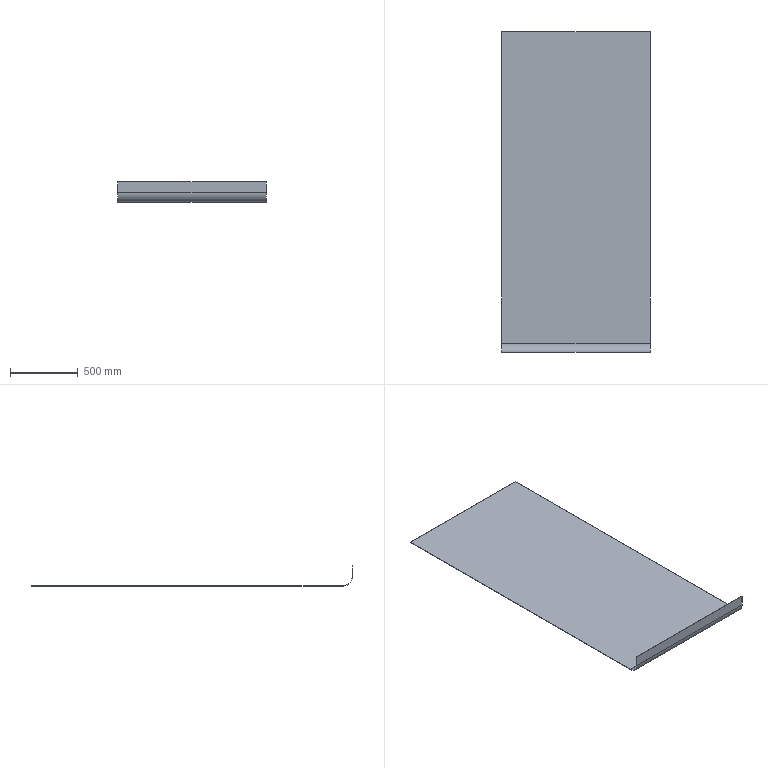Component | SolidWorks | C-SideAluminumHousingAssembly-1_C-SideAluminumCasing1-1 | 1 solid | 14 faces | box 1100 x 2375.5 x 149.5 mm | volume 8226287 mm3 | plane 12 | cylinder 2 | commonest cylinder face diameters 139 x1 133 x1
STEP:
#1=COLOUR_RGB('',0.7922,0.8196,0.9333);
#2=FILL_AREA_STYLE_COLOUR('',#1);
#3=FILL_AREA_STYLE('',(#2));
#4=SURFACE_STYLE_FILL_AREA(#3);
#5=SURFACE_SIDE_STYLE('',(#4));
#6=SURFACE_STYLE_USAGE(.BOTH.,#5);
#7=PRESENTATION_STYLE_ASSIGNMENT((#6));
#8=CARTESIAN_POINT('',(43.307,0.,-0.1181));
#9=VERTEX_POINT('',#8);
#10=CARTESIAN_POINT('',(43.307,0.,0.));
#11=VERTEX_POINT('',#10);
#12=CARTESIAN_POINT('',(43.307,0.,0.));
#13=DIRECTION('',(0.,0.,1.));
#14=VECTOR('',#13,39.37);
#15=LINE('',#12,#14);
#16=EDGE_CURVE('',#9,#11,#15,.T.);
#17=ORIENTED_EDGE('',*,*,#16,.F.);
#18=CARTESIAN_POINT('',(43.307,90.787,-0.1181));
#19=VERTEX_POINT('',#18);
#20=CARTESIAN_POINT('',(43.307,0.,-0.1181));
#21=DIRECTION('',(0.,1.,0.));
#22=VECTOR('',#21,39.37);
#23=LINE('',#20,#22);
#24=EDGE_CURVE('',#9,#19,#23,.T.);
#25=ORIENTED_EDGE('',*,*,#24,.T.);
#26=CARTESIAN_POINT('',(43.307,90.787,0.));
#27=VERTEX_POINT('',#26);
#28=CARTESIAN_POINT('',(43.307,90.787,0.));
#29=DIRECTION('',(0.,0.,1.));
#30=VECTOR('',#29,39.37);
#31=LINE('',#28,#30);
#32=EDGE_CURVE('',#19,#27,#31,.T.);
#33=ORIENTED_EDGE('',*,*,#32,.T.);
#34=CARTESIAN_POINT('',(43.307,0.,0.));
#35=DIRECTION('',(0.,1.,0.));
#36=VECTOR('',#35,39.37);
#37=LINE('',#34,#36);
#38=EDGE_CURVE('',#11,#27,#37,.T.);
#39=ORIENTED_EDGE('',*,*,#38,.F.);
#40=EDGE_LOOP('',(#17,#25,#33,#39));
#41=FACE_OUTER_BOUND('',#40,.T.);
#42=CARTESIAN_POINT('',(43.307,0.,0.));
#43=DIRECTION('',(-1.,0.,0.));
#44=DIRECTION('',(0.,1.,0.));
#45=AXIS2_PLACEMENT_3D('',#42,#43,#44);
#46=PLANE('',#45);
#47=ADVANCED_FACE('',(#41),#46,.F.);
#48=ORIENTED_EDGE('',*,*,#32,.F.);
#49=CARTESIAN_POINT('',(0.,90.787,-0.1181));
#50=VERTEX_POINT('',#49);
#51=CARTESIAN_POINT('',(0.,90.787,-0.1181));
#52=DIRECTION('',(-1.,0.,0.));
#53=VECTOR('',#52,39.37);
#54=LINE('',#51,#53);
#55=EDGE_CURVE('',#19,#50,#54,.T.);
#56=ORIENTED_EDGE('',*,*,#55,.T.);
#57=CARTESIAN_POINT('',(0.,90.787,0.));
#58=VERTEX_POINT('',#57);
#59=CARTESIAN_POINT('',(0.,90.787,0.));
#60=DIRECTION('',(0.,0.,1.));
#61=VECTOR('',#60,39.37);
#62=LINE('',#59,#61);
#63=EDGE_CURVE('',#50,#58,#62,.T.);
#64=ORIENTED_EDGE('',*,*,#63,.T.);
#65=CARTESIAN_POINT('',(0.,90.787,0.));
#66=DIRECTION('',(-1.,0.,0.));
#67=VECTOR('',#66,39.37);
#68=LINE('',#65,#67);
#69=EDGE_CURVE('',#27,#58,#68,.T.);
#70=ORIENTED_EDGE('',*,*,#69,.F.);
#71=EDGE_LOOP('',(#48,#56,#64,#70));
#72=FACE_OUTER_BOUND('',#71,.T.);
#73=CARTESIAN_POINT('',(0.,90.787,0.));
#74=DIRECTION('',(0.,-1.,0.));
#75=DIRECTION('',(-1.,0.,0.));
#76=AXIS2_PLACEMENT_3D('',#73,#74,#75);
#77=PLANE('',#76);
#78=ADVANCED_FACE('',(#72),#77,.F.);
#79=ORIENTED_EDGE('',*,*,#63,.F.);
#80=CARTESIAN_POINT('',(0.,0.,-0.1181));
#81=VERTEX_POINT('',#80);
#82=CARTESIAN_POINT('',(0.,0.,-0.1181));
#83=DIRECTION('',(0.,-1.,0.));
#84=VECTOR('',#83,39.37);
#85=LINE('',#82,#84);
#86=EDGE_CURVE('',#50,#81,#85,.T.);
#87=ORIENTED_EDGE('',*,*,#86,.T.);
#88=CARTESIAN_POINT('',(0.,0.,0.));
#89=VERTEX_POINT('',#88);
#90=CARTESIAN_POINT('',(0.,0.,0.));
#91=DIRECTION('',(0.,0.,1.));
#92=VECTOR('',#91,39.37);
#93=LINE('',#90,#92);
#94=EDGE_CURVE('',#81,#89,#93,.T.);
#95=ORIENTED_EDGE('',*,*,#94,.T.);
#96=CARTESIAN_POINT('',(0.,0.,0.));
#97=DIRECTION('',(0.,-1.,0.));
#98=VECTOR('',#97,39.37);
#99=LINE('',#96,#98);
#100=EDGE_CURVE('',#58,#89,#99,.T.);
#101=ORIENTED_EDGE('',*,*,#100,.F.);
#102=EDGE_LOOP('',(#79,#87,#95,#101));
#103=FACE_OUTER_BOUND('',#102,.T.);
#104=CARTESIAN_POINT('',(0.,0.,0.));
#105=DIRECTION('',(1.,0.,0.));
#106=DIRECTION('',(0.,-1.,0.));
#107=AXIS2_PLACEMENT_3D('',#104,#105,#106);
#108=PLANE('',#107);
#109=ADVANCED_FACE('',(#103),#108,.F.);
#110=ORIENTED_EDGE('',*,*,#100,.T.);
#111=CARTESIAN_POINT('',(0.,0.,0.));
#112=DIRECTION('',(1.,0.,0.));
#113=VECTOR('',#112,39.37);
#114=LINE('',#111,#113);
#115=EDGE_CURVE('',#89,#11,#114,.T.);
#116=ORIENTED_EDGE('',*,*,#115,.T.);
#117=ORIENTED_EDGE('',*,*,#38,.T.);
#118=ORIENTED_EDGE('',*,*,#69,.T.);
#119=EDGE_LOOP('',(#110,#116,#117,#118));
#120=FACE_OUTER_BOUND('',#119,.T.);
#121=CARTESIAN_POINT('',(0.,0.,0.));
#122=DIRECTION('',(0.,0.,-1.));
#123=DIRECTION('',(-1.,0.,0.));
#124=AXIS2_PLACEMENT_3D('',#121,#122,#123);
#125=PLANE('',#124);
#126=ADVANCED_FACE('',(#120),#125,.F.);
#127=ORIENTED_EDGE('',*,*,#86,.F.);
#128=ORIENTED_EDGE('',*,*,#55,.F.);
#129=ORIENTED_EDGE('',*,*,#24,.F.);
#130=CARTESIAN_POINT('',(0.,0.,-0.1181));
#131=DIRECTION('',(1.,0.,0.));
#132=VECTOR('',#131,39.37);
#133=LINE('',#130,#132);
#134=EDGE_CURVE('',#81,#9,#133,.T.);
#135=ORIENTED_EDGE('',*,*,#134,.F.);
#136=EDGE_LOOP('',(#127,#128,#129,#135));
#137=FACE_OUTER_BOUND('',#136,.T.);
#138=CARTESIAN_POINT('',(0.,0.,-0.1181));
#139=DIRECTION('',(0.,0.,-1.));
#140=DIRECTION('',(-1.,0.,0.));
#141=AXIS2_PLACEMENT_3D('',#138,#139,#140);
#142=PLANE('',#141);
#143=ADVANCED_FACE('',(#137),#142,.T.);
#144=CARTESIAN_POINT('',(0.,-2.618,2.618));
#145=VERTEX_POINT('',#144);
#146=CARTESIAN_POINT('',(0.,-2.736,2.618));
#147=VERTEX_POINT('',#146);
#148=CARTESIAN_POINT('',(-0.,-2.736,2.618));
#149=DIRECTION('',(0.,-1.,-0.));
#150=VECTOR('',#149,39.37);
#151=LINE('',#148,#150);
#152=EDGE_CURVE('',#145,#147,#151,.T.);
#153=ORIENTED_EDGE('',*,*,#152,.F.);
#154=CARTESIAN_POINT('',(0.,0.,2.618));
#155=DIRECTION('',(-1.,0.,0.));
#156=DIRECTION('',(0.,0.,-1.));
#157=AXIS2_PLACEMENT_3D('',#154,#155,#156);
#158=CIRCLE('',#157,2.618);
#159=EDGE_CURVE('',#89,#145,#158,.T.);
#160=ORIENTED_EDGE('',*,*,#159,.F.);
#161=ORIENTED_EDGE('',*,*,#94,.F.);
#162=CARTESIAN_POINT('',(0.,0.,2.618));
#163=DIRECTION('',(-1.,0.,0.));
#164=DIRECTION('',(0.,0.,-1.));
#165=AXIS2_PLACEMENT_3D('',#162,#163,#164);
#166=CIRCLE('',#165,2.736);
#167=EDGE_CURVE('',#81,#147,#166,.T.);
#168=ORIENTED_EDGE('',*,*,#167,.T.);
#169=EDGE_LOOP('',(#153,#160,#161,#168));
#170=FACE_OUTER_BOUND('',#169,.T.);
#171=CARTESIAN_POINT('',(0.,0.,2.618));
#172=DIRECTION('',(-1.,0.,0.));
#173=DIRECTION('',(0.,0.,1.));
#174=AXIS2_PLACEMENT_3D('',#171,#172,#173);
#175=PLANE('',#174);
#176=ADVANCED_FACE('',(#170),#175,.T.);
#177=CARTESIAN_POINT('',(43.307,-2.618,2.618));
#178=VERTEX_POINT('',#177);
#179=CARTESIAN_POINT('',(43.307,0.,2.618));
#180=DIRECTION('',(1.,0.,0.));
#181=DIRECTION('',(0.,0.,-1.));
#182=AXIS2_PLACEMENT_3D('',#179,#180,#181);
#183=CIRCLE('',#182,2.618);
#184=EDGE_CURVE('',#178,#11,#183,.T.);
#185=ORIENTED_EDGE('',*,*,#184,.F.);
#186=CARTESIAN_POINT('',(43.307,-2.736,2.618));
#187=VERTEX_POINT('',#186);
#188=CARTESIAN_POINT('',(43.307,-2.618,2.618));
#189=DIRECTION('',(0.,-1.,-0.));
#190=VECTOR('',#189,39.37);
#191=LINE('',#188,#190);
#192=EDGE_CURVE('',#178,#187,#191,.T.);
#193=ORIENTED_EDGE('',*,*,#192,.T.);
#194=CARTESIAN_POINT('',(43.307,0.,2.618));
#195=DIRECTION('',(1.,0.,0.));
#196=DIRECTION('',(0.,0.,-1.));
#197=AXIS2_PLACEMENT_3D('',#194,#195,#196);
#198=CIRCLE('',#197,2.736);
#199=EDGE_CURVE('',#187,#9,#198,.T.);
#200=ORIENTED_EDGE('',*,*,#199,.T.);
#201=ORIENTED_EDGE('',*,*,#16,.T.);
#202=EDGE_LOOP('',(#185,#193,#200,#201));
#203=FACE_OUTER_BOUND('',#202,.T.);
#204=CARTESIAN_POINT('',(43.307,0.,2.618));
#205=DIRECTION('',(-1.,0.,0.));
#206=DIRECTION('',(0.,0.,1.));
#207=AXIS2_PLACEMENT_3D('',#204,#205,#206);
#208=PLANE('',#207);
#209=ADVANCED_FACE('',(#203),#208,.F.);
#210=ORIENTED_EDGE('',*,*,#134,.T.);
#211=ORIENTED_EDGE('',*,*,#199,.F.);
#212=CARTESIAN_POINT('',(0.,-2.736,2.618));
#213=DIRECTION('',(1.,0.,0.));
#214=VECTOR('',#213,39.37);
#215=LINE('',#212,#214);
#216=EDGE_CURVE('',#147,#187,#215,.T.);
#217=ORIENTED_EDGE('',*,*,#216,.F.);
#218=ORIENTED_EDGE('',*,*,#167,.F.);
#219=EDGE_LOOP('',(#210,#211,#217,#218));
#220=FACE_OUTER_BOUND('',#219,.T.);
#221=CARTESIAN_POINT('',(43.307,0.,2.618));
#222=DIRECTION('',(1.,0.,0.));
#223=DIRECTION('',(0.,-1.,-0.));
#224=AXIS2_PLACEMENT_3D('',#221,#222,#223);
#225=CYLINDRICAL_SURFACE('',#224,2.736);
#226=ADVANCED_FACE('',(#220),#225,.T.);
#227=ORIENTED_EDGE('',*,*,#115,.F.);
#228=ORIENTED_EDGE('',*,*,#159,.T.);
#229=CARTESIAN_POINT('',(-0.,-2.618,2.618));
#230=DIRECTION('',(1.,0.,0.));
#231=VECTOR('',#230,39.37);
#232=LINE('',#229,#231);
#233=EDGE_CURVE('',#145,#178,#232,.T.);
#234=ORIENTED_EDGE('',*,*,#233,.T.);
#235=ORIENTED_EDGE('',*,*,#184,.T.);
#236=EDGE_LOOP('',(#227,#228,#234,#235));
#237=FACE_OUTER_BOUND('',#236,.T.);
#238=CARTESIAN_POINT('',(43.307,0.,2.618));
#239=DIRECTION('',(1.,0.,0.));
#240=DIRECTION('',(0.,-1.,-0.));
#241=AXIS2_PLACEMENT_3D('',#238,#239,#240);
#242=CYLINDRICAL_SURFACE('',#241,2.618);
#243=ADVANCED_FACE('',(#237),#242,.F.);
#244=CARTESIAN_POINT('',(43.307,-2.736,5.768));
#245=VERTEX_POINT('',#244);
#246=CARTESIAN_POINT('',(43.307,-2.736,-0.));
#247=DIRECTION('',(0.,0.,-1.));
#248=VECTOR('',#247,39.37);
#249=LINE('',#246,#248);
#250=EDGE_CURVE('',#245,#187,#249,.T.);
#251=ORIENTED_EDGE('',*,*,#250,.T.);
#252=ORIENTED_EDGE('',*,*,#192,.F.);
#253=CARTESIAN_POINT('',(43.307,-2.618,5.768));
#254=VERTEX_POINT('',#253);
#255=CARTESIAN_POINT('',(43.307,-2.618,0.));
#256=DIRECTION('',(0.,0.,-1.));
#257=VECTOR('',#256,39.37);
#258=LINE('',#255,#257);
#259=EDGE_CURVE('',#254,#178,#258,.T.);
#260=ORIENTED_EDGE('',*,*,#259,.F.);
#261=CARTESIAN_POINT('',(43.307,-2.736,5.768));
#262=DIRECTION('',(0.,1.,0.));
#263=VECTOR('',#262,39.37);
#264=LINE('',#261,#263);
#265=EDGE_CURVE('',#245,#254,#264,.T.);
#266=ORIENTED_EDGE('',*,*,#265,.F.);
#267=EDGE_LOOP('',(#251,#252,#260,#266));
#268=FACE_OUTER_BOUND('',#267,.T.);
#269=CARTESIAN_POINT('',(43.307,-2.736,-0.));
#270=DIRECTION('',(1.,0.,0.));
#271=DIRECTION('',(0.,0.,-1.));
#272=AXIS2_PLACEMENT_3D('',#269,#270,#271);
#273=PLANE('',#272);
#274=ADVANCED_FACE('',(#268),#273,.T.);
#275=CARTESIAN_POINT('',(-0.,-2.618,5.768));
#276=VERTEX_POINT('',#275);
#277=CARTESIAN_POINT('',(0.,-2.618,0.));
#278=DIRECTION('',(-0.,-0.,1.));
#279=VECTOR('',#278,39.37);
#280=LINE('',#277,#279);
#281=EDGE_CURVE('',#145,#276,#280,.T.);
#282=ORIENTED_EDGE('',*,*,#281,.F.);
#283=ORIENTED_EDGE('',*,*,#152,.T.);
#284=CARTESIAN_POINT('',(-0.,-2.736,5.768));
#285=VERTEX_POINT('',#284);
#286=CARTESIAN_POINT('',(-0.,-2.736,5.768));
#287=DIRECTION('',(-0.,-0.,1.));
#288=VECTOR('',#287,39.37);
#289=LINE('',#286,#288);
#290=EDGE_CURVE('',#147,#285,#289,.T.);
#291=ORIENTED_EDGE('',*,*,#290,.T.);
#292=CARTESIAN_POINT('',(-0.,-2.736,5.768));
#293=DIRECTION('',(0.,1.,0.));
#294=VECTOR('',#293,39.37);
#295=LINE('',#292,#294);
#296=EDGE_CURVE('',#285,#276,#295,.T.);
#297=ORIENTED_EDGE('',*,*,#296,.T.);
#298=EDGE_LOOP('',(#282,#283,#291,#297));
#299=FACE_OUTER_BOUND('',#298,.T.);
#300=CARTESIAN_POINT('',(-0.,-2.736,5.768));
#301=DIRECTION('',(-1.,0.,-0.));
#302=DIRECTION('',(-0.,0.,1.));
#303=AXIS2_PLACEMENT_3D('',#300,#301,#302);
#304=PLANE('',#303);
#305=ADVANCED_FACE('',(#299),#304,.T.);
#306=ORIENTED_EDGE('',*,*,#290,.F.);
#307=ORIENTED_EDGE('',*,*,#216,.T.);
#308=ORIENTED_EDGE('',*,*,#250,.F.);
#309=CARTESIAN_POINT('',(43.307,-2.736,5.768));
#310=DIRECTION('',(1.,0.,0.));
#311=VECTOR('',#310,39.37);
#312=LINE('',#309,#311);
#313=EDGE_CURVE('',#285,#245,#312,.T.);
#314=ORIENTED_EDGE('',*,*,#313,.F.);
#315=EDGE_LOOP('',(#306,#307,#308,#314));
#316=FACE_OUTER_BOUND('',#315,.T.);
#317=CARTESIAN_POINT('',(0.,-2.736,-0.));
#318=DIRECTION('',(0.,-1.,-0.));
#319=DIRECTION('',(0.,0.,-1.));
#320=AXIS2_PLACEMENT_3D('',#317,#318,#319);
#321=PLANE('',#320);
#322=ADVANCED_FACE('',(#316),#321,.T.);
#323=ORIENTED_EDGE('',*,*,#233,.F.);
#324=ORIENTED_EDGE('',*,*,#281,.T.);
#325=CARTESIAN_POINT('',(0.,-2.618,5.768));
#326=DIRECTION('',(1.,0.,0.));
#327=VECTOR('',#326,39.37);
#328=LINE('',#325,#327);
#329=EDGE_CURVE('',#276,#254,#328,.T.);
#330=ORIENTED_EDGE('',*,*,#329,.T.);
#331=ORIENTED_EDGE('',*,*,#259,.T.);
#332=EDGE_LOOP('',(#323,#324,#330,#331));
#333=FACE_OUTER_BOUND('',#332,.T.);
#334=CARTESIAN_POINT('',(0.,-2.618,0.));
#335=DIRECTION('',(0.,-1.,-0.));
#336=DIRECTION('',(0.,0.,-1.));
#337=AXIS2_PLACEMENT_3D('',#334,#335,#336);
#338=PLANE('',#337);
#339=ADVANCED_FACE('',(#333),#338,.F.);
#340=ORIENTED_EDGE('',*,*,#329,.F.);
#341=ORIENTED_EDGE('',*,*,#296,.F.);
#342=ORIENTED_EDGE('',*,*,#313,.T.);
#343=ORIENTED_EDGE('',*,*,#265,.T.);
#344=EDGE_LOOP('',(#340,#341,#342,#343));
#345=FACE_OUTER_BOUND('',#344,.T.);
#346=CARTESIAN_POINT('',(43.307,-2.736,5.768));
#347=DIRECTION('',(0.,-0.,1.));
#348=DIRECTION('',(0.,-1.,-0.));
#349=AXIS2_PLACEMENT_3D('',#346,#347,#348);
#350=PLANE('',#349);
#351=ADVANCED_FACE('',(#345),#350,.T.);
#352=CLOSED_SHELL('',(#47,#78,#109,#126,#143,#176,#209,#226,#243,#274,#305,#322,#339,#351));
#353=MANIFOLD_SOLID_BREP('',#352);
#354=STYLED_ITEM('',(#7),#353);
#355=PRESENTATION_LAYER_ASSIGNMENT('','',(#354));
#356=(LENGTH_UNIT()NAMED_UNIT(*)SI_UNIT($,.METRE.));
#357=LENGTH_MEASURE_WITH_UNIT(LENGTH_MEASURE(0.0254),#356);
#358=DIMENSIONAL_EXPONENTS(1.,0.,0.,0.,0.,0.,0.);
#359=(CONVERSION_BASED_UNIT('',#357)LENGTH_UNIT()NAMED_UNIT(#358));
#360=UNCERTAINTY_MEASURE_WITH_UNIT(LENGTH_MEASURE(0.00001),#359,'','');
#361=(NAMED_UNIT(*)PLANE_ANGLE_UNIT()SI_UNIT($,.RADIAN.));
#362=(NAMED_UNIT(*)SI_UNIT($,.STERADIAN.)SOLID_ANGLE_UNIT());
#363=(GEOMETRIC_REPRESENTATION_CONTEXT(3)GLOBAL_UNCERTAINTY_ASSIGNED_CONTEXT((#360))GLOBAL_UNIT_ASSIGNED_CONTEXT((#359,#361,#362))REPRESENTATION_CONTEXT('',''));
#364=MECHANICAL_DESIGN_GEOMETRIC_PRESENTATION_REPRESENTATION('',(#354),#363);
#365=CARTESIAN_POINT('',(0.,0.,0.));
#366=DIRECTION('',(0.,0.,1.));
#367=DIRECTION('',(1.,0.,0.));
#368=AXIS2_PLACEMENT_3D('',#365,#366,#367);
#369=(LENGTH_UNIT()NAMED_UNIT(*)SI_UNIT($,.METRE.));
#370=LENGTH_MEASURE_WITH_UNIT(LENGTH_MEASURE(0.0254),#369);
#371=DIMENSIONAL_EXPONENTS(1.,0.,0.,0.,0.,0.,0.);
#372=(CONVERSION_BASED_UNIT('',#370)LENGTH_UNIT()NAMED_UNIT(#371));
#373=UNCERTAINTY_MEASURE_WITH_UNIT(LENGTH_MEASURE(0.00001),#372,'','');
#374=(NAMED_UNIT(*)PLANE_ANGLE_UNIT()SI_UNIT($,.RADIAN.));
#375=(NAMED_UNIT(*)SI_UNIT($,.STERADIAN.)SOLID_ANGLE_UNIT());
#376=(GEOMETRIC_REPRESENTATION_CONTEXT(3)GLOBAL_UNCERTAINTY_ASSIGNED_CONTEXT((#373))GLOBAL_UNIT_ASSIGNED_CONTEXT((#372,#374,#375))REPRESENTATION_CONTEXT('',''));
#377=ADVANCED_BREP_SHAPE_REPRESENTATION('',(#353,#368),#376);